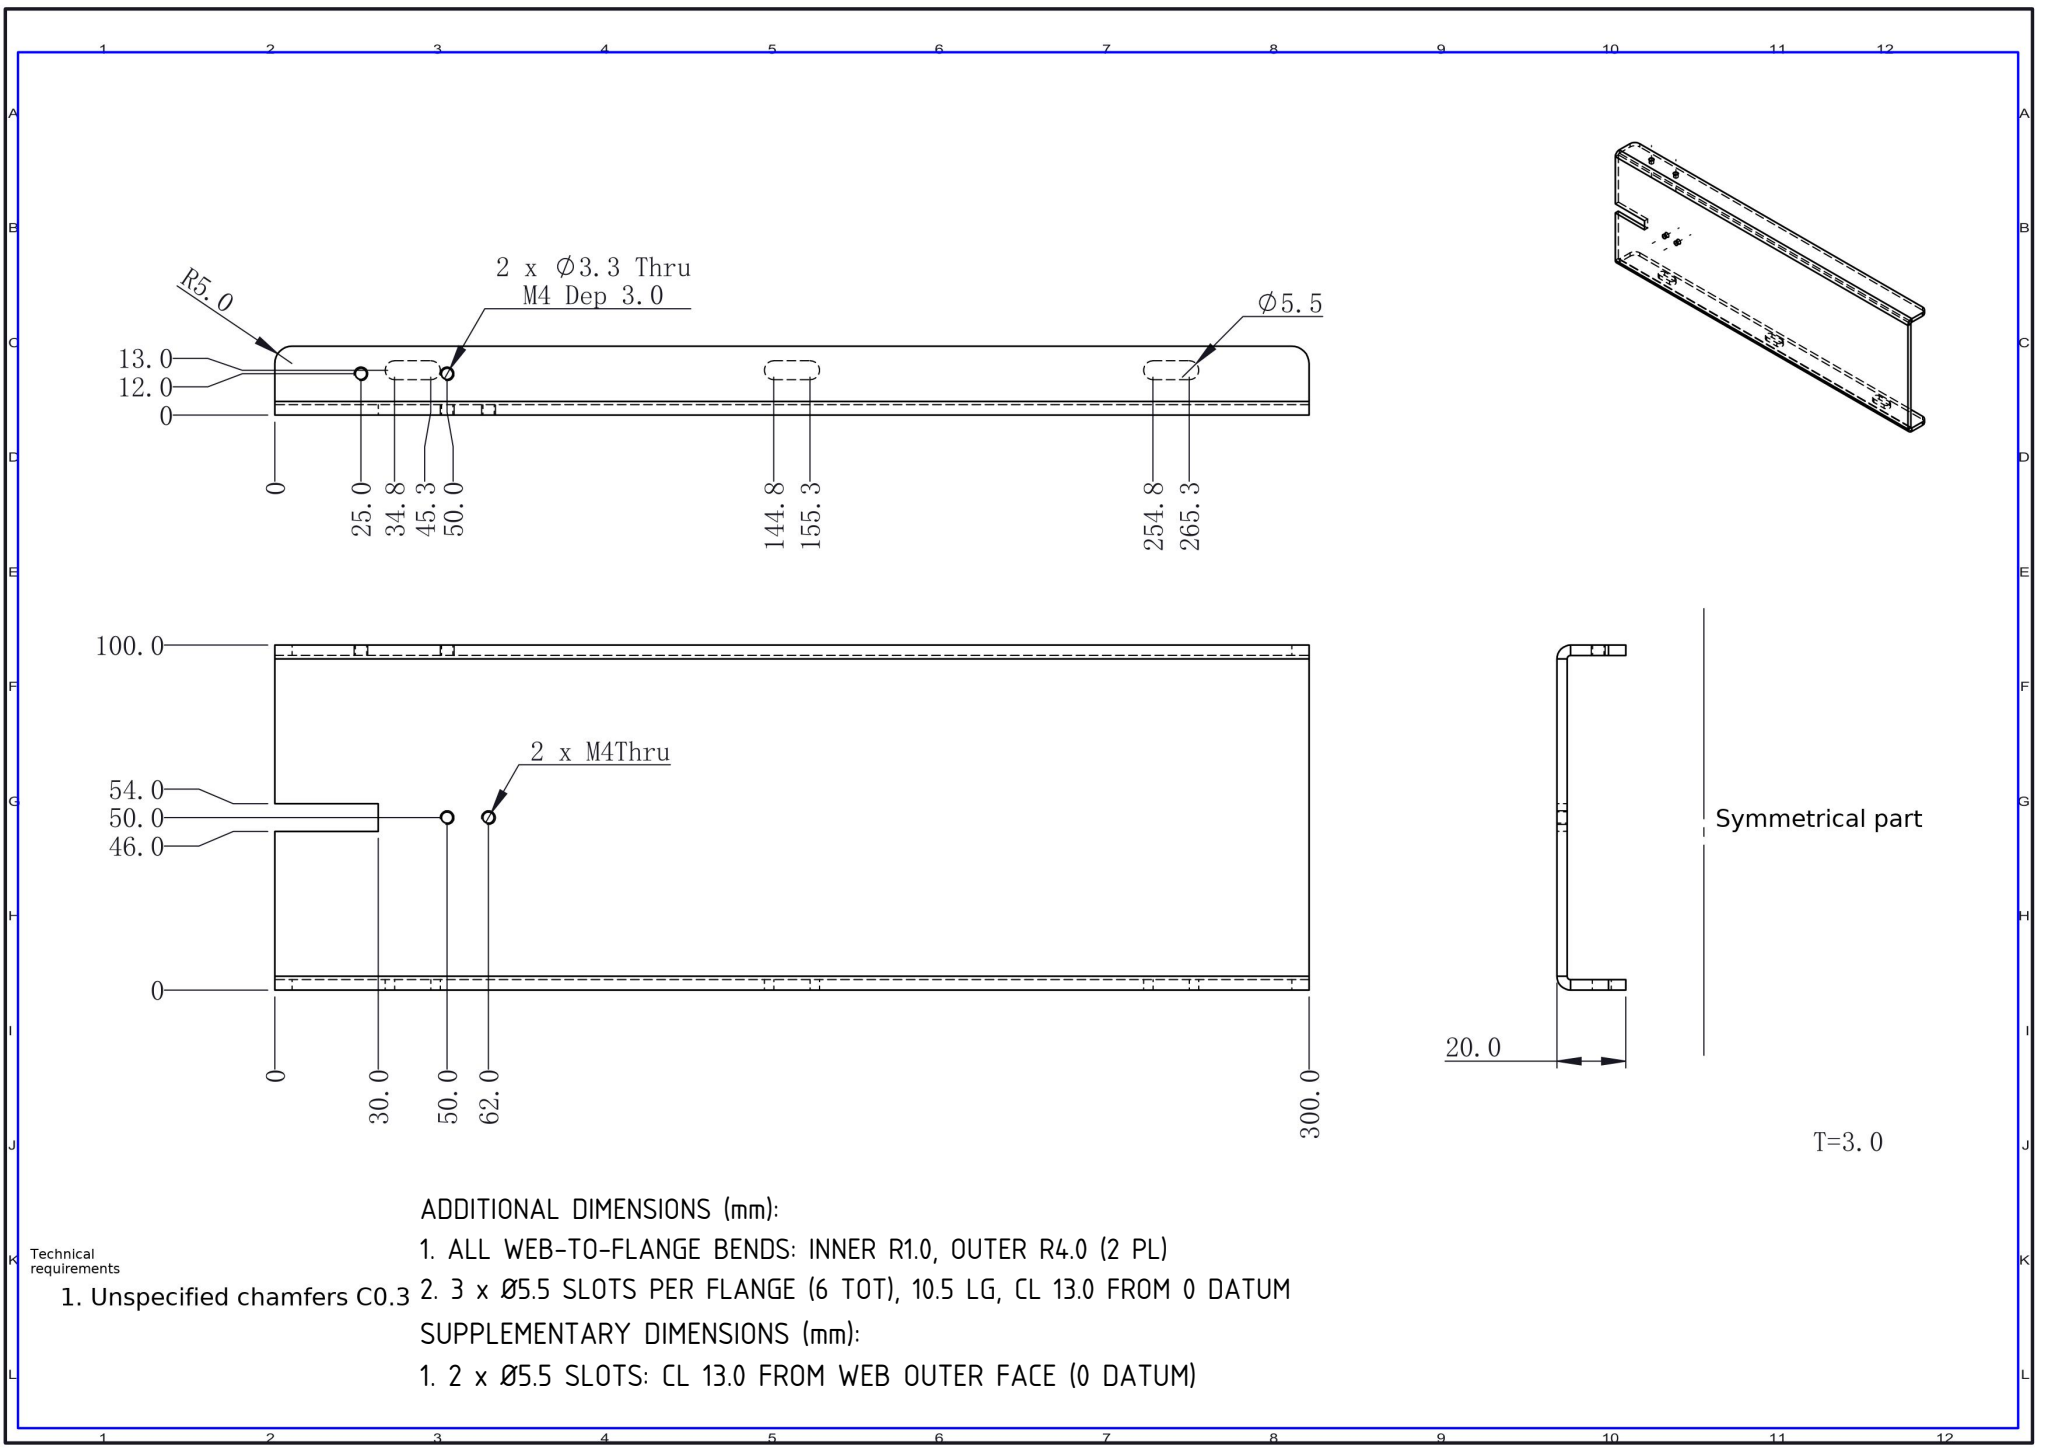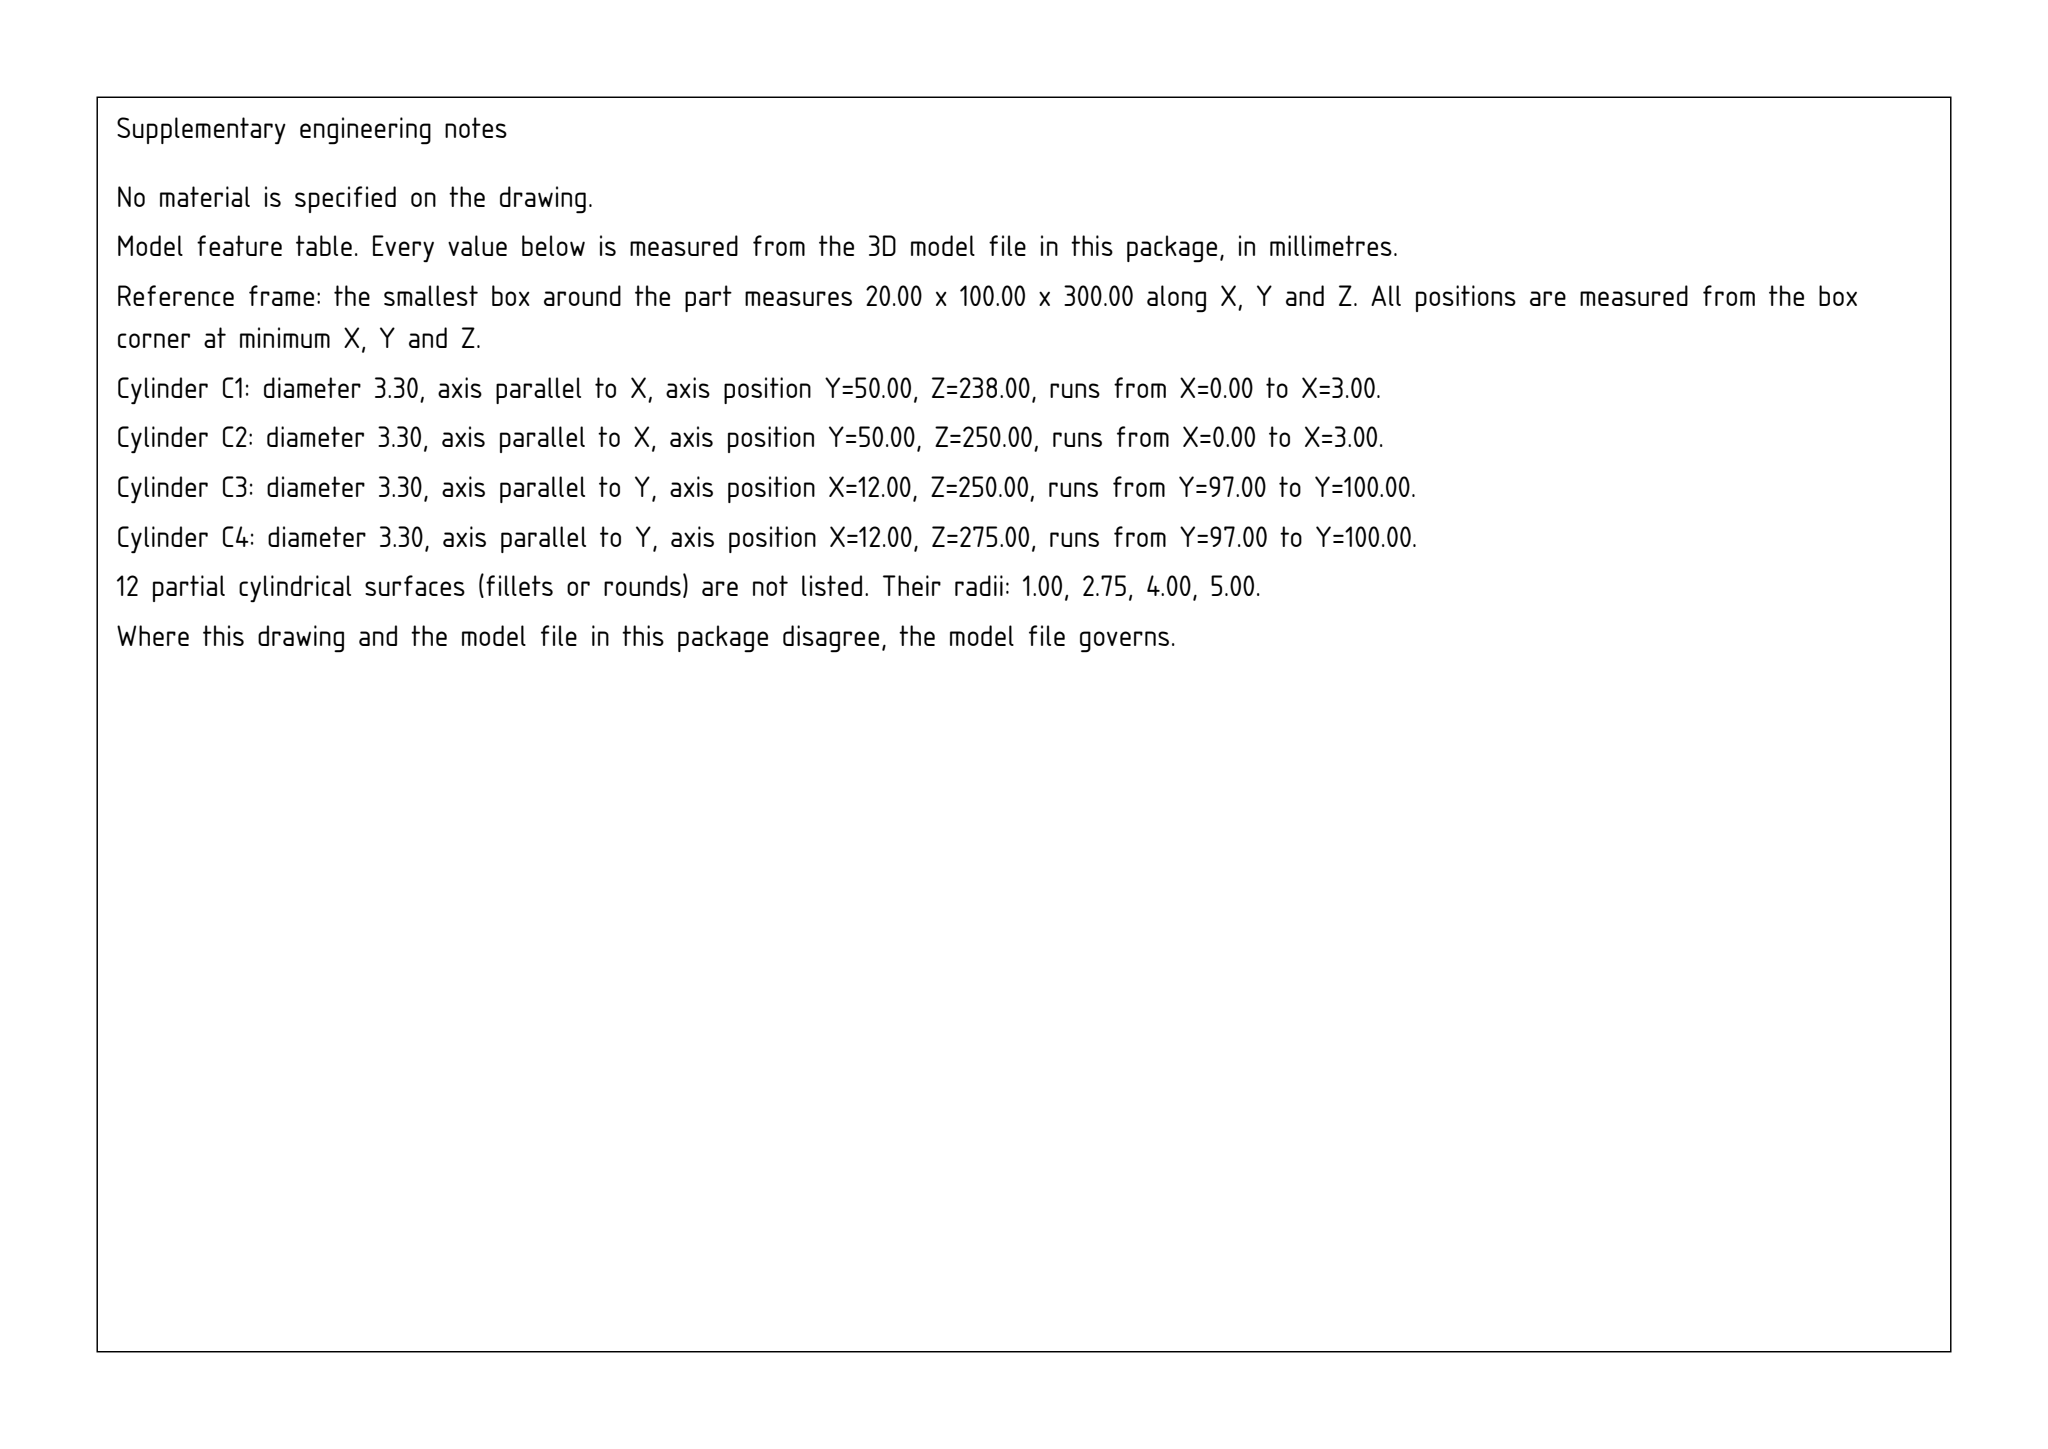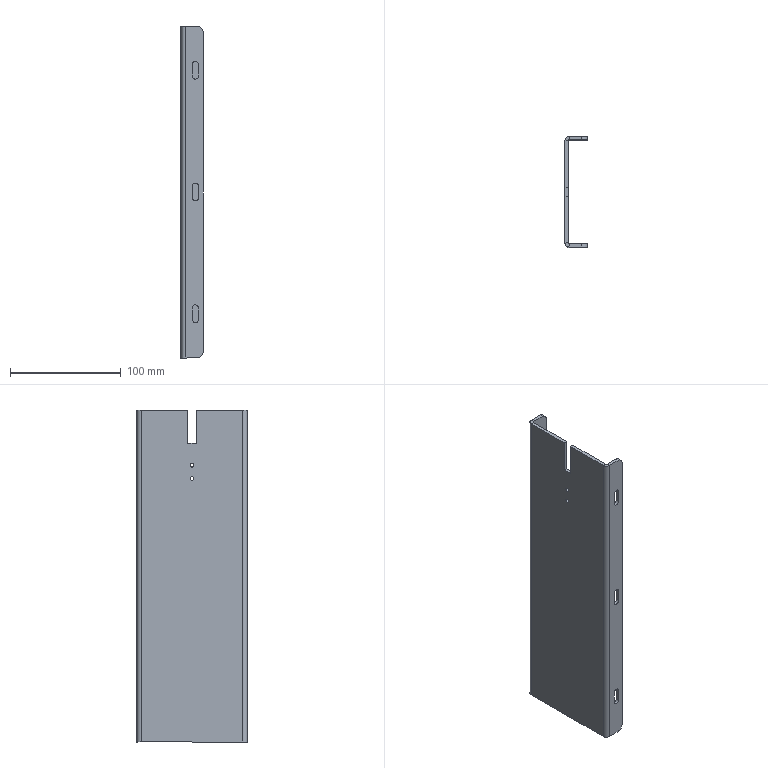Part | SolidWorks | mm | 1 solid | 53 faces | box 20 x 100 x 300 mm | volume 117048 mm3 | plane 28 | cylinder 25 | commonest cylinder face diameters 5.5 x9 3.3 x8 10 x4 8 x2 2 x2